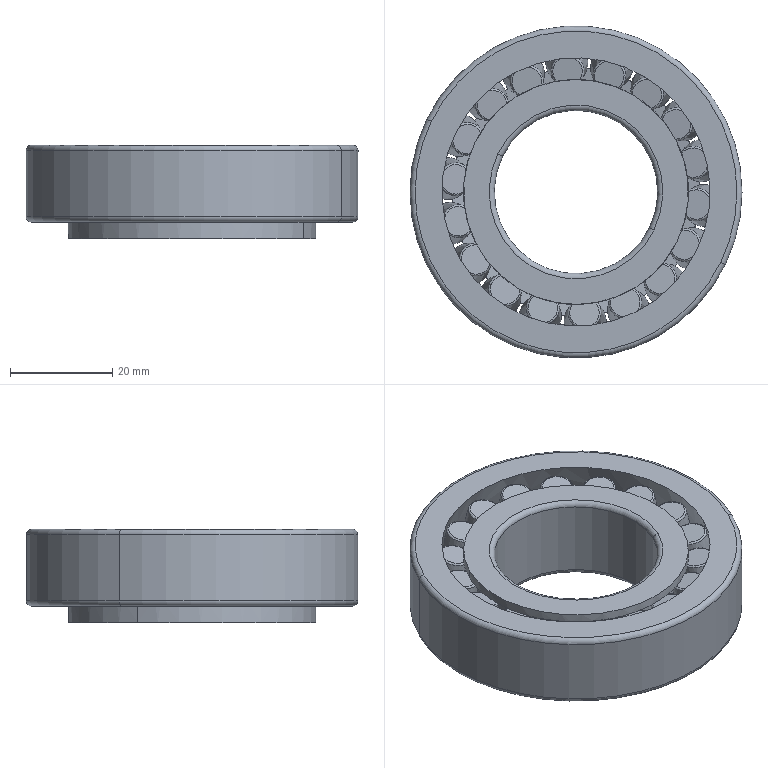Component | SolidWorks | PartAssemblyInLowerHousing-1_LowSpeedAxisAssembly-1_tapered roller bearings gb-4 | 1 solid | 172 faces | volume 32654 mm3 | torus 80 | cone 44 | plane 40 | cylinder 8 | commonest cylinder face diameters 65 x2 44.025 x2 48.5 x2 32 x2